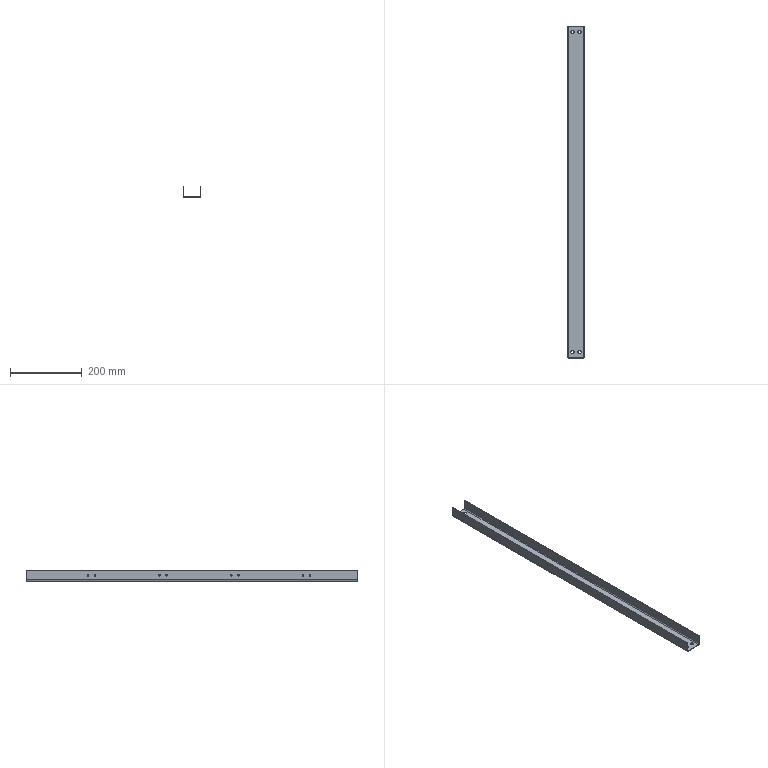Component | SolidWorks | FrameLongitudinalBeamFour01100-1 | 1 solid | 66 faces | volume 144129 mm3 | cylinder 48 | plane 18 | commonest cylinder face diameters 4.5 x32 9 x8 6 x4 8 x2 5 x2